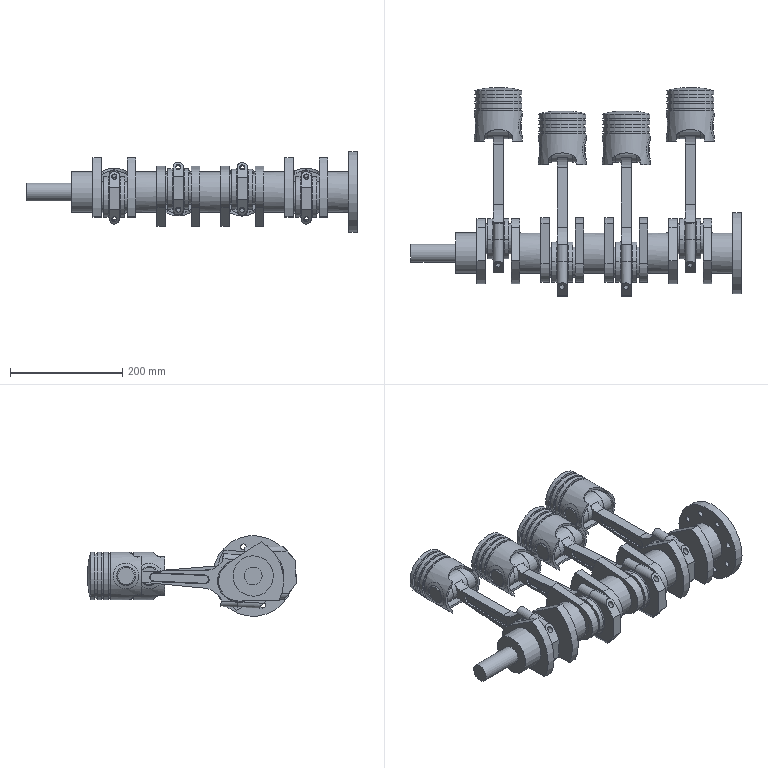Assembly | NX | mm | 17 component files | 21 solids | 522 faces | box 589 x 371.54 x 144 mm | volume 4288102 mm3 | cylinder 246 | plane 224 | torus 32 | cone 16 | spline 4 | commonest cylinder face diameters 72 x29 85 x16 33.8 x16 20 x16 80 x16 6 x16 54 x16 18 x16
Bill of materials:
unnamed part 1 | 4 |  | Hollow, thin-walled cylindrical body with a slightly domed closed end, three circumferential grooves near that end, and two coaxial round holes through opposite sides of the wall. Internal bosses surround the holes, and arched cutouts are cut into the open skirt end. The overall form resembles a piston.
unnamed part 2 | 4 |  | Solid plain cylinder with flat end faces and a small chamfer around both end edges. It resembles a pin or dowel.
unnamed part 3 | 4 |  | Elongated link with a closed round eye at one end and an open half-circle saddle at the other. A tapered beam joins them, with a shallow elongated pocket recessed into its side face. Two bolt-hole lugs flank the half-bore. The overall form resembles a connecting rod body without its cap.
unnamed part 4 | 1 |  | Long multi-throw shaft. It has a small-diameter stub at one end and a large circular flange at the other. Along its length it carries a series of cylindrical journals separated by plate-like webs, with some cylindrical sections offset from the main axis. The flange face has a ring of small holes. The overall form resembles a crankshaft.
unnamed part 5 | 4 |  | Half-ring cap block with a semicircular bore. A stepped or relief band runs around the bore, and the outer back has angled chamfered faces. Two eared lugs with through-holes sit on either side of the bore opening. The shape resembles a connecting-rod or bearing cap.
Mates:
1. touch align | 7_CRANKSHAFT 1 face | assembly line
2. touch align | 7_CRANKSHAFT 1 face | assembly datumplane
3. touch align | 2_PISTON_HEAD 1 face | assembly line
4. touch align | 2_PISTON_HEAD 2 face | assembly line
5. touch align | 2_PISTON_HEAD 4 face | assembly line
6. touch align | 2_PISTON_HEAD 3 face | assembly line
7. touch align | 4_CONNECTING_ROD 1 face | 7_CRANKSHAFT 1 face
8. touch align | 4_CONNECTING_ROD 2 face | 7_CRANKSHAFT 1 face
9. touch align | 4_CONNECTING_ROD 3 face | 7_CRANKSHAFT 1 face
10. touch align | 4_CONNECTING_ROD 4 face | 7_CRANKSHAFT 1 face
11. touch align | 4_CONNECTING_ROD 1 face | 2_PISTON_HEAD 1 face
12. touch align | 4_CONNECTING_ROD 3 face | 2_PISTON_HEAD 4 face
13. touch align | 4_CONNECTING_ROD 4 face | 2_PISTON_HEAD 3 face
14. touch align | 4_CONNECTING_ROD 2 face | 2_PISTON_HEAD 2 face
15. touch align | 5_CONNECTING_ROD_CAP 1 face | 4_CONNECTING_ROD 1 face
16. touch align | 5_CONNECTING_ROD_CAP 2 face | 4_CONNECTING_ROD 2 face
17. touch align | 5_CONNECTING_ROD_CAP 4 face | 4_CONNECTING_ROD 3 face
18. touch align | 5_CONNECTING_ROD_CAP 3 face | 4_CONNECTING_ROD 4 face
19. touch align | 5_CONNECTING_ROD_CAP 1 face | 4_CONNECTING_ROD 1 face
20. touch align | 5_CONNECTING_ROD_CAP 2 face | 4_CONNECTING_ROD 2 face
21. touch align | 5_CONNECTING_ROD_CAP 4 face | 4_CONNECTING_ROD 3 face
22. touch align | 5_CONNECTING_ROD_CAP 3 face | 4_CONNECTING_ROD 4 face
23. touch align | 5_CONNECTING_ROD_CAP 3 face | 4_CONNECTING_ROD 4 face
24. touch align | 5_CONNECTING_ROD_CAP 4 face | 4_CONNECTING_ROD 3 face
25. touch align | 5_CONNECTING_ROD_CAP 2 face | 4_CONNECTING_ROD 2 face
26. touch align | 5_CONNECTING_ROD_CAP 1 face | 4_CONNECTING_ROD 1 face
27. touch align | 4_CONNECTING_ROD 1 face | 2_PISTON_HEAD 1 face
28. touch align | 4_CONNECTING_ROD 2 face | 2_PISTON_HEAD 2 face
29. touch align | 4_CONNECTING_ROD 3 face | 2_PISTON_HEAD 4 face
30. touch align | 4_CONNECTING_ROD 4 face | 2_PISTON_HEAD 3 face
31. touch align | 6_PISTON_PIN 3 face | 2_PISTON_HEAD 1 face
32. center | 6_PISTON_PIN 3 face | 6_PISTON_PIN 3 face | 2_PISTON_HEAD 1 face
33. touch align | 6_PISTON_PIN 2 face | 2_PISTON_HEAD 2 face
34. center | 6_PISTON_PIN 2 face | 6_PISTON_PIN 2 face | 2_PISTON_HEAD 2 face
35. touch align | 6_PISTON_PIN 4 face | 2_PISTON_HEAD 4 face
36. center | 6_PISTON_PIN 4 face | 6_PISTON_PIN 4 face | 2_PISTON_HEAD 4 face
37. touch align | 6_PISTON_PIN 1 face | 2_PISTON_HEAD 3 face
38. center | 6_PISTON_PIN 1 face | 6_PISTON_PIN 1 face | 2_PISTON_HEAD 3 face